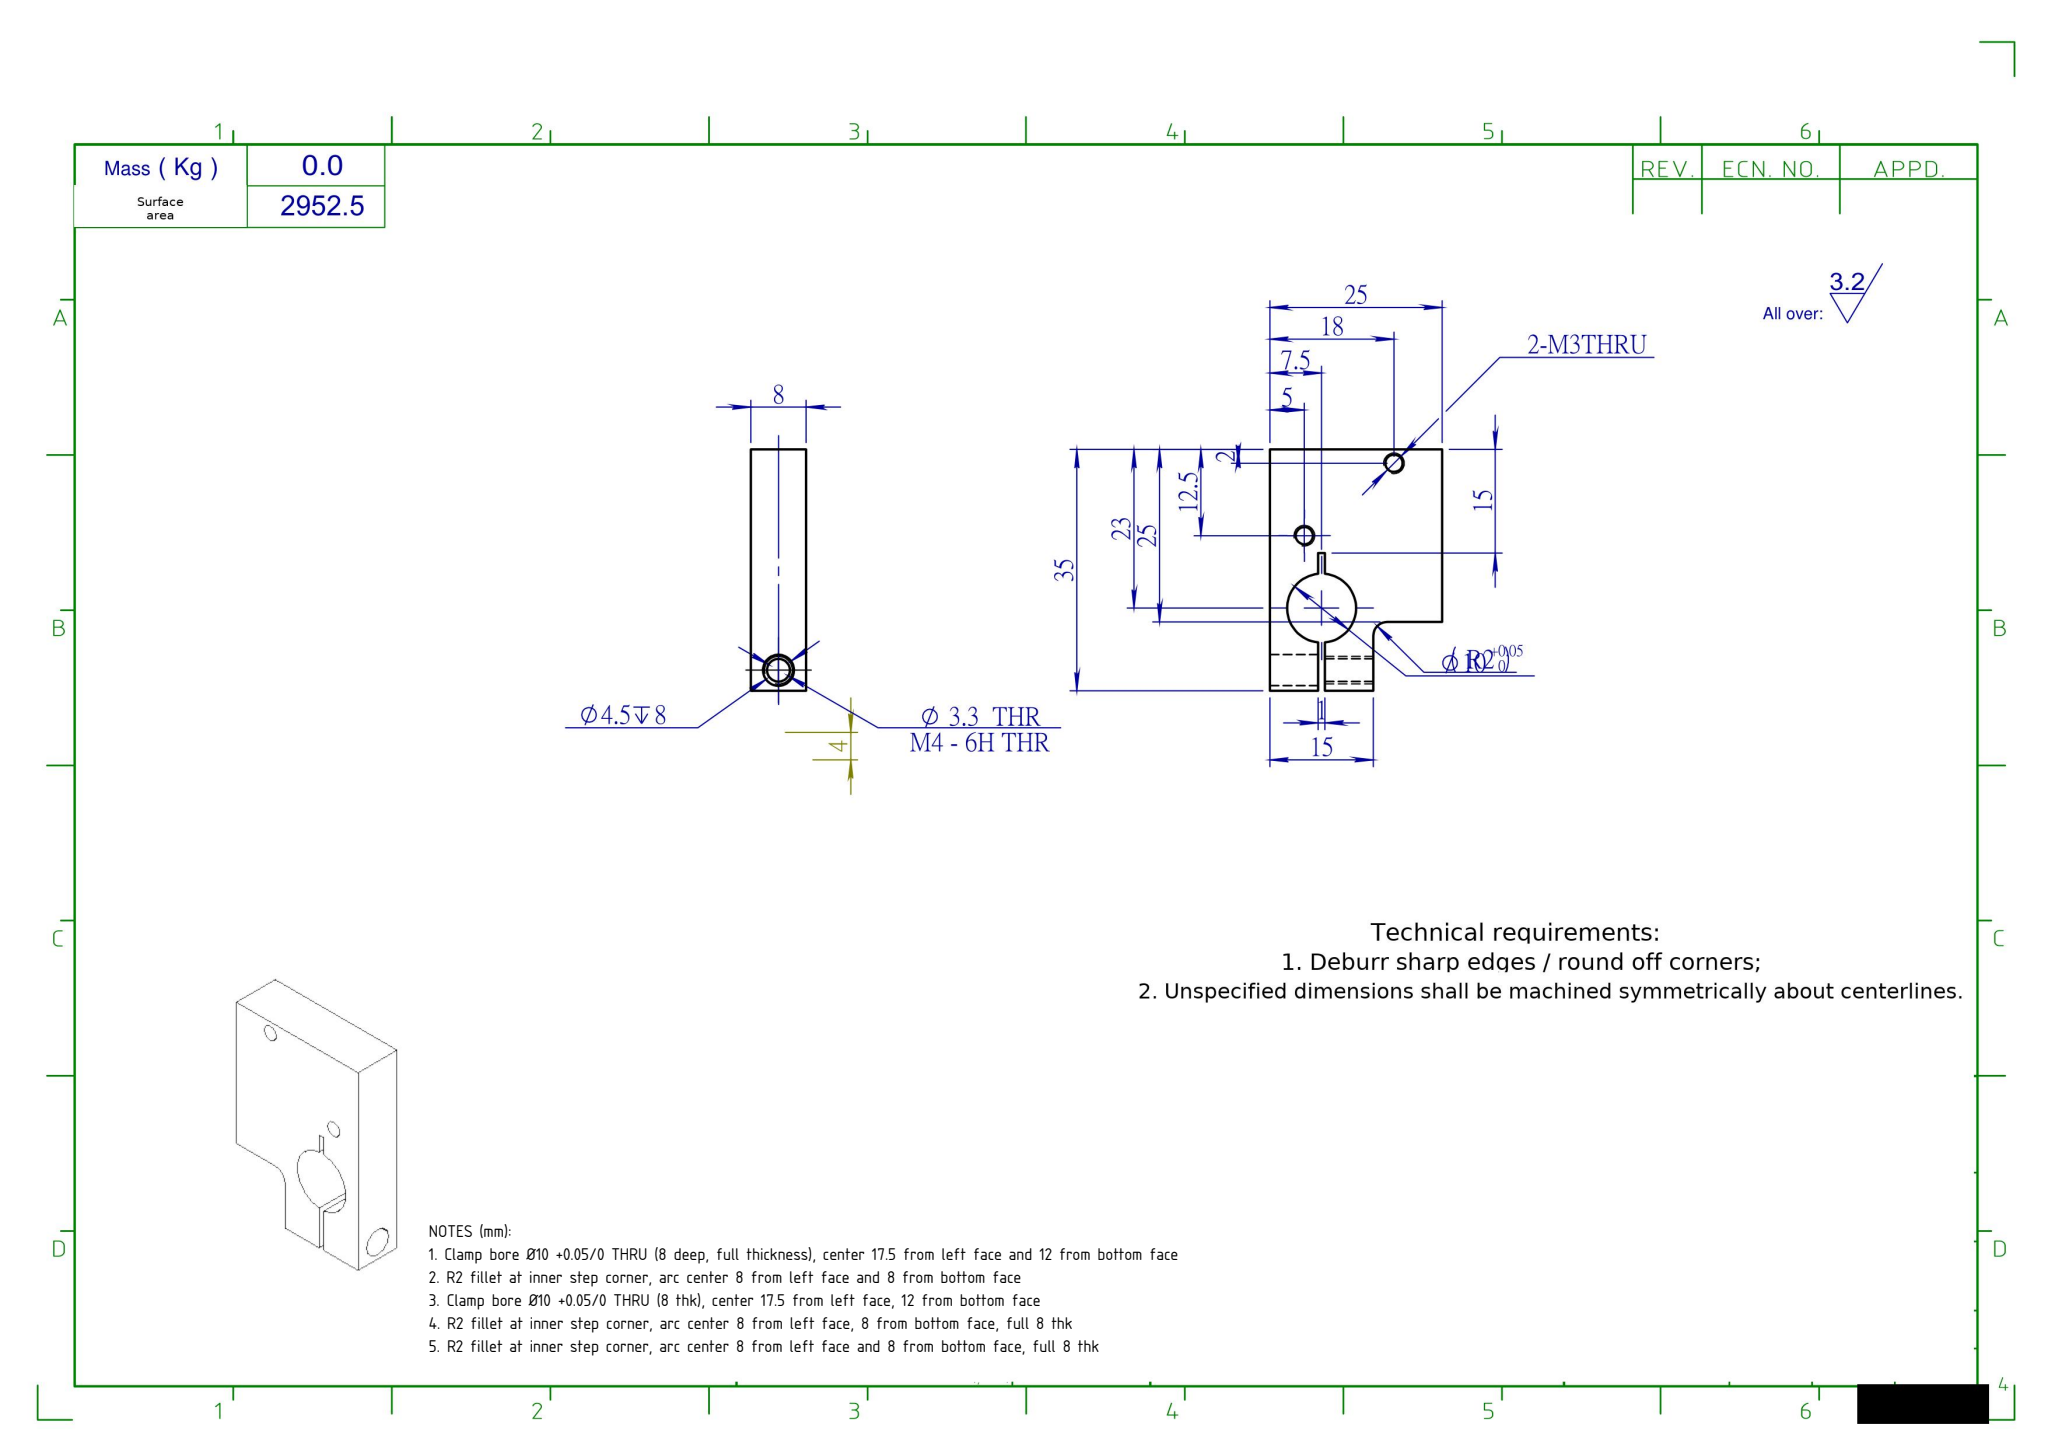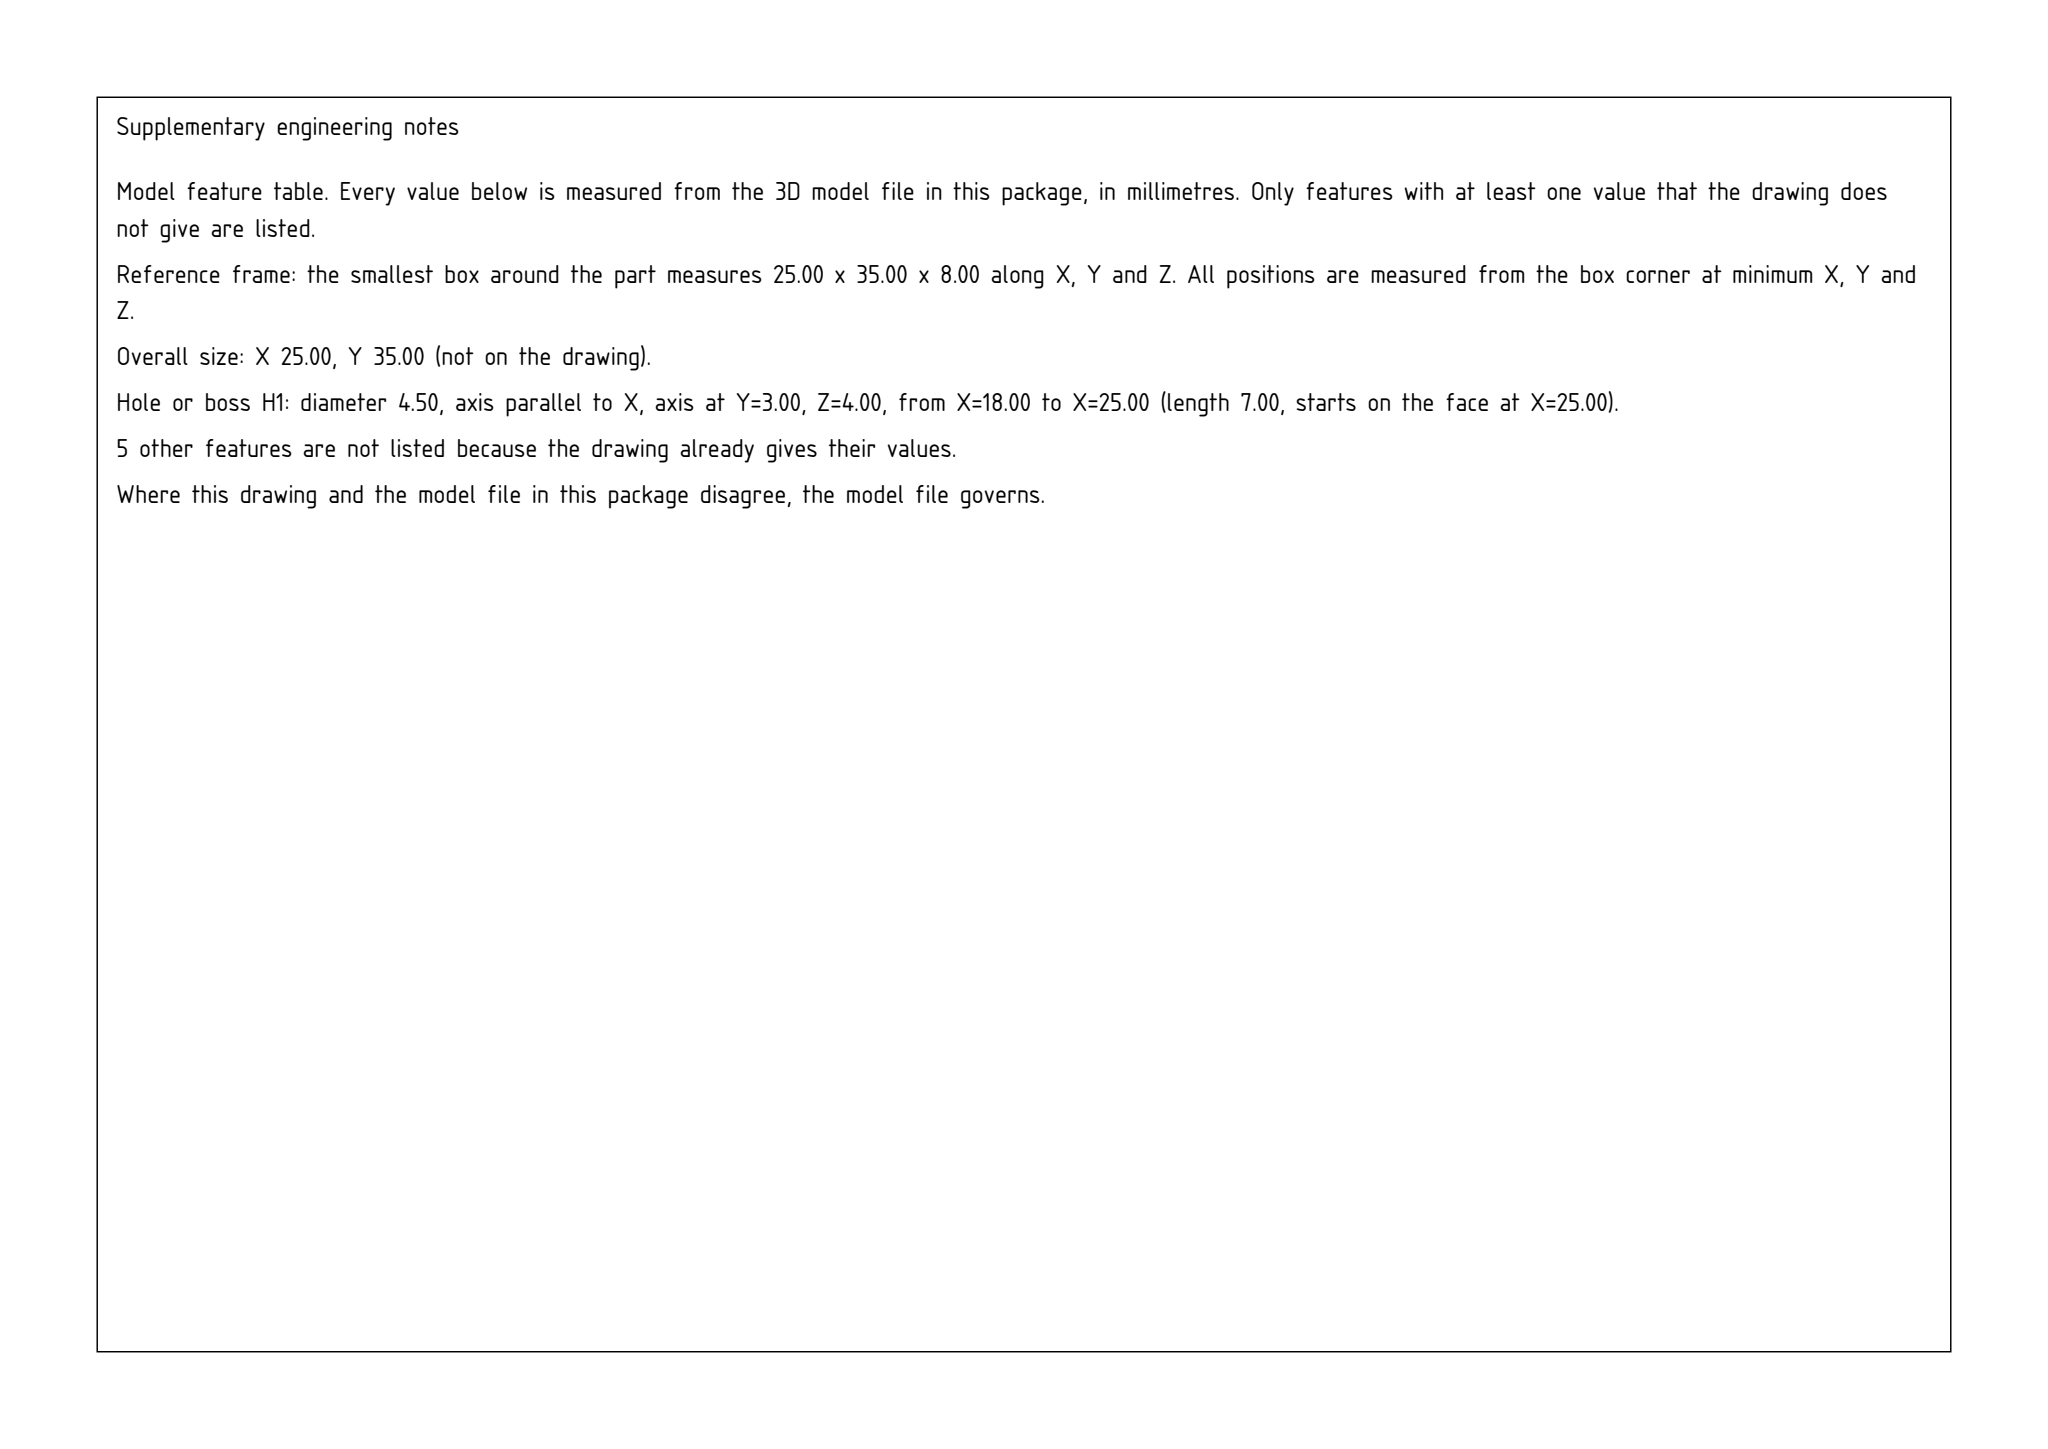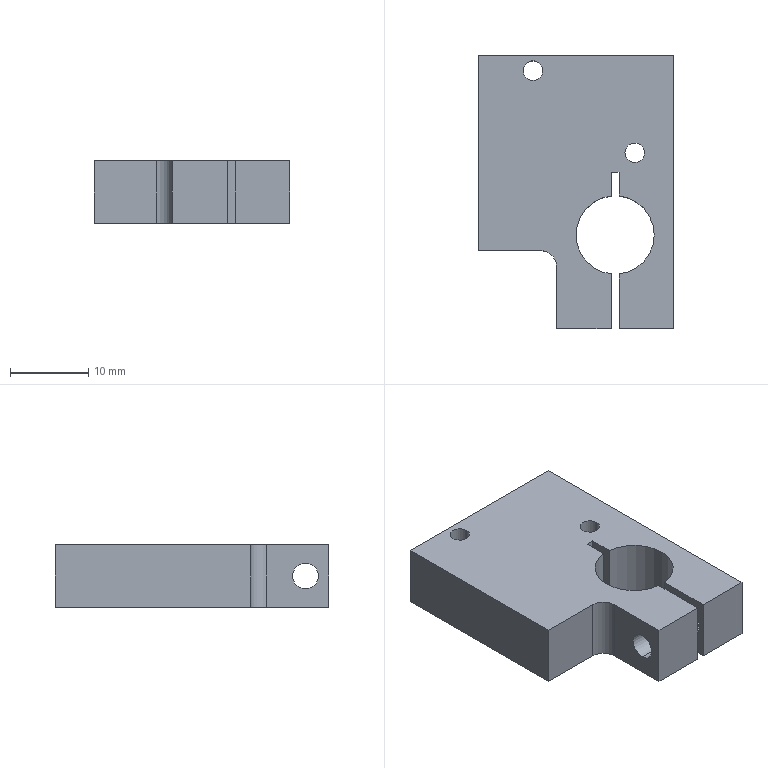Part | SolidWorks | mm | 1 solid | 26 faces | box 25 x 35 x 8 mm | volume 5249 mm3 | plane 14 | cylinder 12 | commonest cylinder face diameters 2.5 x4 10 x3 3.3 x2 4.5 x2 4 x1
Drawing notes:
Clamp bore Ø10 +0.05/0 THRU (8 deep, full thickness), center 17.5 from left face and 12 from bottom face | from the solid: cylinders: concave arc dia 10.0, axis z at [17.5, 12.0], from z0 to z8 (337° open to slot)
R2 fillet at inner step corner, arc center 8 from left face and 8 from bottom face | from the solid: cylinders: concave arc dia 4.0, axis z at [8.0, 8.0], from z0 to z8, arc 90°
Clamp bore Ø10 +0.05/0 THRU (8 thk), center 17.5 from left face, 12 from bottom face | from the solid: cylinders: concave arc dia 10.0, axis z at [17.5, 12.0], from 0.0 to 8.0
R2 fillet at inner step corner, arc center 8 from left face, 8 from bottom face, full 8 thk | from the solid: cylinders: concave arc dia 4.0 (R2), axis z at [8.0, 8.0], 90 deg, from 0.0 to 8.0
R2 fillet at inner step corner, arc center 8 from left face and 8 from bottom face, full 8 thk | from the solid: cylinders: concave arc dia 4.0 (R2), axis z at (8.0, 8.0), from 0.0 to 8.0 (90 deg)
build123d program:
from build123d import *

# Parameters (mm, degrees)
SKETCH1_W          = 15
SKETCH1_H          = 35
EXTRUDE1_DEPTH     = 8
SKETCH2_R          = 5
CUT_EXTRUDE1_DEPTH = 10
SKETCH3_W          = 1
SKETCH3_H          = 20
CUT_EXTRUDE2_DEPTH = 10
SKETCH8_W          = 8
SKETCH8_H          = 25
EXTRUDE2_DEPTH     = 10
SKETCH9_R          = 2.25
CUT_EXTRUDE3_DEPTH = 8
M4_TAPPED_HOLE1_D  = 3.3
M3_TAPPED_HOLE6_D  = 2.5
FILLET1_R          = 2


with BuildPart() as part:
    # Sketch1 → Extrude1 (new body)
    with BuildSketch(Plane.XY):
        with Locations((-14.432, 24.37)):
            Rectangle(SKETCH1_W, SKETCH1_H)
    extrude(amount=EXTRUDE1_DEPTH)

    # Sketch2 → Cut-Extrude1 (cut)
    with BuildSketch(Plane(origin=(0, 0, 0), x_dir=(-1, 0, 0), z_dir=(0, 0, -1))):
        with Locations((14.432, 18.87)):
            Circle(SKETCH2_R)
    extrude(amount=-CUT_EXTRUDE1_DEPTH, mode=Mode.SUBTRACT)

    # Sketch3 → Cut-Extrude2 (cut)
    with BuildSketch(Plane(origin=(0, 0, 0), x_dir=(-1, 0, 0), z_dir=(0, 0, -1))):
        with Locations((14.432, 16.87)):
            Rectangle(SKETCH3_W, SKETCH3_H)
    extrude(amount=-CUT_EXTRUDE2_DEPTH, mode=Mode.SUBTRACT)

    # Sketch8 → Extrude2 (add)
    with BuildSketch(Plane.ZY.offset(21.932)):
        with Locations((4, 29.37)):
            Rectangle(SKETCH8_W, SKETCH8_H)
    extrude(amount=EXTRUDE2_DEPTH)

    # Sketch9 → Cut-Extrude3 (cut)
    with BuildSketch(Plane.ZY.offset(6.932)):
        with Locations(Location((4, 9.87, 0), (0, 0, 90))):
            Circle(SKETCH9_R)
    extrude(amount=CUT_EXTRUDE3_DEPTH, mode=Mode.SUBTRACT)

    # M4 Tapped Hole1 (through all)
    with Locations(Plane(origin=(-14.932, -11.083, 0.1076), x_dir=(0, 0, 1), z_dir=(1, 0, 0))):
        with Locations((3.892, -20.953)):
            Hole(M4_TAPPED_HOLE1_D / 2)

    # M3 Tapped Hole6 (through all)
    with Locations(Plane(origin=(0, 0, 0), x_dir=(-1, 0, 0), z_dir=(0, 0, -1))):
        with Locations((11.932, 29.37), (24.932, 39.87)):
            Hole(M3_TAPPED_HOLE6_D / 2)

    # Fillet1
    fillet1_edges = [part.edges().sort_by_distance(p)[0] for p in [
        (-21.932, 16.87, 4),
    ]]
    fillet(fillet1_edges, radius=FILLET1_R)


solid = part.part
STEP:
#1=CARTESIAN_POINT('',(-13.182,29.37,8.));
#2=VERTEX_POINT('',#1);
#3=CARTESIAN_POINT('',(-10.682,29.37,8.));
#4=VERTEX_POINT('',#3);
#5=CARTESIAN_POINT('',(-11.932,29.37,8.));
#6=DIRECTION('',(0.,0.,1.));
#7=DIRECTION('',(1.,0.,0.));
#8=AXIS2_PLACEMENT_3D('',#5,#6,#7);
#9=CIRCLE('',#8,1.25);
#10=EDGE_CURVE('',#2,#4,#9,.T.);
#11=ORIENTED_EDGE('',*,*,#10,.T.);
#12=CARTESIAN_POINT('',(-10.682,29.37,-0.));
#13=VERTEX_POINT('',#12);
#14=CARTESIAN_POINT('',(-10.682,29.37,0.));
#15=DIRECTION('',(0.,0.,-1.));
#16=VECTOR('',#15,1000.);
#17=LINE('',#14,#16);
#18=EDGE_CURVE('',#4,#13,#17,.T.);
#19=ORIENTED_EDGE('',*,*,#18,.T.);
#20=CARTESIAN_POINT('',(-13.182,29.37,-0.));
#21=VERTEX_POINT('',#20);
#22=CARTESIAN_POINT('',(-11.932,29.37,-0.));
#23=DIRECTION('',(0.,0.,-1.));
#24=DIRECTION('',(-1.,0.,0.));
#25=AXIS2_PLACEMENT_3D('',#22,#23,#24);
#26=CIRCLE('',#25,1.25);
#27=EDGE_CURVE('',#13,#21,#26,.T.);
#28=ORIENTED_EDGE('',*,*,#27,.T.);
#29=CARTESIAN_POINT('',(-13.182,29.37,0.));
#30=DIRECTION('',(0.,0.,-1.));
#31=VECTOR('',#30,1000.);
#32=LINE('',#29,#31);
#33=EDGE_CURVE('',#2,#21,#32,.T.);
#34=ORIENTED_EDGE('',*,*,#33,.F.);
#35=EDGE_LOOP('',(#11,#19,#28,#34));
#36=FACE_OUTER_BOUND('',#35,.T.);
#37=CARTESIAN_POINT('',(-11.932,29.37,0.));
#38=DIRECTION('',(0.,0.,-1.));
#39=DIRECTION('',(-1.,0.,0.));
#40=AXIS2_PLACEMENT_3D('',#37,#38,#39);
#41=CYLINDRICAL_SURFACE('',#40,1.25);
#42=ADVANCED_FACE('',(#36),#41,.F.);
#43=CARTESIAN_POINT('',(-26.182,39.87,8.));
#44=VERTEX_POINT('',#43);
#45=CARTESIAN_POINT('',(-23.682,39.87,8.));
#46=VERTEX_POINT('',#45);
#47=CARTESIAN_POINT('',(-24.932,39.87,8.));
#48=DIRECTION('',(0.,0.,1.));
#49=DIRECTION('',(1.,0.,0.));
#50=AXIS2_PLACEMENT_3D('',#47,#48,#49);
#51=CIRCLE('',#50,1.25);
#52=EDGE_CURVE('',#44,#46,#51,.T.);
#53=ORIENTED_EDGE('',*,*,#52,.T.);
#54=CARTESIAN_POINT('',(-23.682,39.87,-0.));
#55=VERTEX_POINT('',#54);
#56=CARTESIAN_POINT('',(-23.682,39.87,0.));
#57=DIRECTION('',(0.,0.,-1.));
#58=VECTOR('',#57,1000.);
#59=LINE('',#56,#58);
#60=EDGE_CURVE('',#46,#55,#59,.T.);
#61=ORIENTED_EDGE('',*,*,#60,.T.);
#62=CARTESIAN_POINT('',(-26.182,39.87,-0.));
#63=VERTEX_POINT('',#62);
#64=CARTESIAN_POINT('',(-24.932,39.87,-0.));
#65=DIRECTION('',(0.,0.,-1.));
#66=DIRECTION('',(-1.,0.,0.));
#67=AXIS2_PLACEMENT_3D('',#64,#65,#66);
#68=CIRCLE('',#67,1.25);
#69=EDGE_CURVE('',#55,#63,#68,.T.);
#70=ORIENTED_EDGE('',*,*,#69,.T.);
#71=CARTESIAN_POINT('',(-26.182,39.87,0.));
#72=DIRECTION('',(0.,0.,-1.));
#73=VECTOR('',#72,1000.);
#74=LINE('',#71,#73);
#75=EDGE_CURVE('',#44,#63,#74,.T.);
#76=ORIENTED_EDGE('',*,*,#75,.F.);
#77=EDGE_LOOP('',(#53,#61,#70,#76));
#78=FACE_OUTER_BOUND('',#77,.T.);
#79=CARTESIAN_POINT('',(-24.932,39.87,0.));
#80=DIRECTION('',(0.,0.,-1.));
#81=DIRECTION('',(-1.,0.,0.));
#82=AXIS2_PLACEMENT_3D('',#79,#80,#81);
#83=CYLINDRICAL_SURFACE('',#82,1.25);
#84=ADVANCED_FACE('',(#78),#83,.F.);
#85=CARTESIAN_POINT('',(-21.932,9.87,5.65));
#86=VERTEX_POINT('',#85);
#87=CARTESIAN_POINT('',(-21.932,9.87,2.35));
#88=VERTEX_POINT('',#87);
#89=CARTESIAN_POINT('',(-21.932,9.87,4.));
#90=DIRECTION('',(1.,0.,0.));
#91=DIRECTION('',(0.,1.,0.));
#92=AXIS2_PLACEMENT_3D('',#89,#90,#91);
#93=CIRCLE('',#92,1.65);
#94=EDGE_CURVE('',#86,#88,#93,.T.);
#95=ORIENTED_EDGE('',*,*,#94,.F.);
#96=CARTESIAN_POINT('',(-14.932,9.87,5.65));
#97=VERTEX_POINT('',#96);
#98=CARTESIAN_POINT('',(-14.932,9.87,5.65));
#99=DIRECTION('',(1.,0.,0.));
#100=VECTOR('',#99,1000.);
#101=LINE('',#98,#100);
#102=EDGE_CURVE('',#86,#97,#101,.T.);
#103=ORIENTED_EDGE('',*,*,#102,.T.);
#104=CARTESIAN_POINT('',(-14.932,9.87,2.35));
#105=VERTEX_POINT('',#104);
#106=CARTESIAN_POINT('',(-14.932,9.87,4.));
#107=DIRECTION('',(1.,0.,0.));
#108=DIRECTION('',(0.,0.,-1.));
#109=AXIS2_PLACEMENT_3D('',#106,#107,#108);
#110=CIRCLE('',#109,1.65);
#111=EDGE_CURVE('',#97,#105,#110,.T.);
#112=ORIENTED_EDGE('',*,*,#111,.T.);
#113=CARTESIAN_POINT('',(-14.932,9.87,2.35));
#114=DIRECTION('',(1.,0.,0.));
#115=VECTOR('',#114,1000.);
#116=LINE('',#113,#115);
#117=EDGE_CURVE('',#88,#105,#116,.T.);
#118=ORIENTED_EDGE('',*,*,#117,.F.);
#119=EDGE_LOOP('',(#95,#103,#112,#118));
#120=FACE_OUTER_BOUND('',#119,.T.);
#121=CARTESIAN_POINT('',(-14.932,9.87,4.));
#122=DIRECTION('',(1.,0.,0.));
#123=DIRECTION('',(0.,0.,-1.));
#124=AXIS2_PLACEMENT_3D('',#121,#122,#123);
#125=CYLINDRICAL_SURFACE('',#124,1.65);
#126=ADVANCED_FACE('',(#120),#125,.F.);
#127=CARTESIAN_POINT('',(-13.932,12.12,4.));
#128=VERTEX_POINT('',#127);
#129=CARTESIAN_POINT('',(-13.932,7.62,4.));
#130=VERTEX_POINT('',#129);
#131=CARTESIAN_POINT('',(-13.932,9.87,4.));
#132=DIRECTION('',(-1.,0.,0.));
#133=DIRECTION('',(0.,1.,0.));
#134=AXIS2_PLACEMENT_3D('',#131,#132,#133);
#135=CIRCLE('',#134,2.25);
#136=EDGE_CURVE('',#128,#130,#135,.T.);
#137=ORIENTED_EDGE('',*,*,#136,.T.);
#138=CARTESIAN_POINT('',(-6.932,7.62,4.));
#139=VERTEX_POINT('',#138);
#140=CARTESIAN_POINT('',(-14.932,7.62,4.));
#141=DIRECTION('',(1.,0.,0.));
#142=VECTOR('',#141,1000.);
#143=LINE('',#140,#142);
#144=EDGE_CURVE('',#130,#139,#143,.T.);
#145=ORIENTED_EDGE('',*,*,#144,.T.);
#146=CARTESIAN_POINT('',(-6.932,12.12,4.));
#147=VERTEX_POINT('',#146);
#148=CARTESIAN_POINT('',(-6.932,9.87,4.));
#149=DIRECTION('',(-1.,-0.,0.));
#150=DIRECTION('',(0.,-1.,0.));
#151=AXIS2_PLACEMENT_3D('',#148,#149,#150);
#152=CIRCLE('',#151,2.25);
#153=EDGE_CURVE('',#147,#139,#152,.T.);
#154=ORIENTED_EDGE('',*,*,#153,.F.);
#155=CARTESIAN_POINT('',(-14.932,12.12,4.));
#156=DIRECTION('',(1.,0.,0.));
#157=VECTOR('',#156,1000.);
#158=LINE('',#155,#157);
#159=EDGE_CURVE('',#128,#147,#158,.T.);
#160=ORIENTED_EDGE('',*,*,#159,.F.);
#161=EDGE_LOOP('',(#137,#145,#154,#160));
#162=FACE_OUTER_BOUND('',#161,.T.);
#163=CARTESIAN_POINT('',(-14.932,9.87,4.));
#164=DIRECTION('',(1.,0.,0.));
#165=DIRECTION('',(0.,1.,0.));
#166=AXIS2_PLACEMENT_3D('',#163,#164,#165);
#167=CYLINDRICAL_SURFACE('',#166,2.25);
#168=ADVANCED_FACE('',(#162),#167,.F.);
#169=CARTESIAN_POINT('',(-14.932,23.845,8.));
#170=VERTEX_POINT('',#169);
#171=CARTESIAN_POINT('',(-19.432,18.87,8.));
#172=VERTEX_POINT('',#171);
#173=CARTESIAN_POINT('',(-14.432,18.87,8.));
#174=DIRECTION('',(0.,0.,1.));
#175=DIRECTION('',(1.,0.,0.));
#176=AXIS2_PLACEMENT_3D('',#173,#174,#175);
#177=CIRCLE('',#176,5.);
#178=EDGE_CURVE('',#170,#172,#177,.T.);
#179=ORIENTED_EDGE('',*,*,#178,.T.);
#180=CARTESIAN_POINT('',(-19.432,18.87,0.));
#181=VERTEX_POINT('',#180);
#182=CARTESIAN_POINT('',(-19.432,18.87,10.));
#183=DIRECTION('',(0.,0.,-1.));
#184=VECTOR('',#183,1000.);
#185=LINE('',#182,#184);
#186=EDGE_CURVE('',#172,#181,#185,.T.);
#187=ORIENTED_EDGE('',*,*,#186,.T.);
#188=CARTESIAN_POINT('',(-14.932,23.845,0.));
#189=VERTEX_POINT('',#188);
#190=CARTESIAN_POINT('',(-14.432,18.87,0.));
#191=DIRECTION('',(0.,0.,-1.));
#192=DIRECTION('',(-1.,0.,0.));
#193=AXIS2_PLACEMENT_3D('',#190,#191,#192);
#194=CIRCLE('',#193,5.);
#195=EDGE_CURVE('',#181,#189,#194,.T.);
#196=ORIENTED_EDGE('',*,*,#195,.T.);
#197=CARTESIAN_POINT('',(-14.932,23.845,10.));
#198=DIRECTION('',(0.,0.,1.));
#199=VECTOR('',#198,1000.);
#200=LINE('',#197,#199);
#201=EDGE_CURVE('',#189,#170,#200,.T.);
#202=ORIENTED_EDGE('',*,*,#201,.T.);
#203=EDGE_LOOP('',(#179,#187,#196,#202));
#204=FACE_OUTER_BOUND('',#203,.T.);
#205=CARTESIAN_POINT('',(-14.432,18.87,10.));
#206=DIRECTION('',(0.,0.,-1.));
#207=DIRECTION('',(-1.,0.,0.));
#208=AXIS2_PLACEMENT_3D('',#205,#206,#207);
#209=CYLINDRICAL_SURFACE('',#208,5.);
#210=ADVANCED_FACE('',(#204),#209,.F.);
#211=CARTESIAN_POINT('',(-6.932,6.87,0.));
#212=VERTEX_POINT('',#211);
#213=CARTESIAN_POINT('',(-6.932,41.87,0.));
#214=VERTEX_POINT('',#213);
#215=CARTESIAN_POINT('',(-6.932,41.87,0.));
#216=DIRECTION('',(-0.,1.,0.));
#217=VECTOR('',#216,1000.);
#218=LINE('',#215,#217);
#219=EDGE_CURVE('',#212,#214,#218,.T.);
#220=ORIENTED_EDGE('',*,*,#219,.T.);
#221=CARTESIAN_POINT('',(-6.932,41.87,8.));
#222=VERTEX_POINT('',#221);
#223=CARTESIAN_POINT('',(-6.932,41.87,8.));
#224=DIRECTION('',(0.,0.,-1.));
#225=VECTOR('',#224,1000.);
#226=LINE('',#223,#225);
#227=EDGE_CURVE('',#222,#214,#226,.T.);
#228=ORIENTED_EDGE('',*,*,#227,.F.);
#229=CARTESIAN_POINT('',(-6.932,6.87,8.));
#230=VERTEX_POINT('',#229);
#231=CARTESIAN_POINT('',(-6.932,41.87,8.));
#232=DIRECTION('',(-0.,1.,0.));
#233=VECTOR('',#232,1000.);
#234=LINE('',#231,#233);
#235=EDGE_CURVE('',#230,#222,#234,.T.);
#236=ORIENTED_EDGE('',*,*,#235,.F.);
#237=CARTESIAN_POINT('',(-6.932,6.87,8.));
#238=DIRECTION('',(0.,0.,-1.));
#239=VECTOR('',#238,1000.);
#240=LINE('',#237,#239);
#241=EDGE_CURVE('',#230,#212,#240,.T.);
#242=ORIENTED_EDGE('',*,*,#241,.T.);
#243=EDGE_LOOP('',(#220,#228,#236,#242));
#244=FACE_OUTER_BOUND('',#243,.T.);
#245=ORIENTED_EDGE('',*,*,#153,.T.);
#246=CARTESIAN_POINT('',(-6.932,9.87,4.));
#247=DIRECTION('',(-1.,-0.,0.));
#248=DIRECTION('',(0.,-1.,0.));
#249=AXIS2_PLACEMENT_3D('',#246,#247,#248);
#250=CIRCLE('',#249,2.25);
#251=EDGE_CURVE('',#139,#147,#250,.T.);
#252=ORIENTED_EDGE('',*,*,#251,.T.);
#253=EDGE_LOOP('',(#245,#252));
#254=FACE_BOUND('',#253,.T.);
#255=CARTESIAN_POINT('',(-6.932,41.87,8.));
#256=DIRECTION('',(-1.,-0.,0.));
#257=DIRECTION('',(0.,-1.,0.));
#258=AXIS2_PLACEMENT_3D('',#255,#256,#257);
#259=PLANE('',#258);
#260=ADVANCED_FACE('',(#244,#254),#259,.F.);
#261=CARTESIAN_POINT('',(-13.932,6.87,8.));
#262=VERTEX_POINT('',#261);
#263=CARTESIAN_POINT('',(-13.932,13.895,8.));
#264=VERTEX_POINT('',#263);
#265=CARTESIAN_POINT('',(-13.932,6.87,8.));
#266=DIRECTION('',(0.,1.,0.));
#267=VECTOR('',#266,1000.);
#268=LINE('',#265,#267);
#269=EDGE_CURVE('',#262,#264,#268,.T.);
#270=ORIENTED_EDGE('',*,*,#269,.T.);
#271=CARTESIAN_POINT('',(-13.932,13.895,0.));
#272=VERTEX_POINT('',#271);
#273=CARTESIAN_POINT('',(-13.932,13.895,10.));
#274=DIRECTION('',(0.,0.,1.));
#275=VECTOR('',#274,1000.);
#276=LINE('',#273,#275);
#277=EDGE_CURVE('',#272,#264,#276,.T.);
#278=ORIENTED_EDGE('',*,*,#277,.F.);
#279=CARTESIAN_POINT('',(-13.932,6.87,0.));
#280=VERTEX_POINT('',#279);
#281=CARTESIAN_POINT('',(-13.932,26.87,0.));
#282=DIRECTION('',(-0.,-1.,0.));
#283=VECTOR('',#282,1000.);
#284=LINE('',#281,#283);
#285=EDGE_CURVE('',#272,#280,#284,.T.);
#286=ORIENTED_EDGE('',*,*,#285,.T.);
#287=CARTESIAN_POINT('',(-13.932,6.87,10.));
#288=DIRECTION('',(0.,0.,-1.));
#289=VECTOR('',#288,1000.);
#290=LINE('',#287,#289);
#291=EDGE_CURVE('',#262,#280,#290,.T.);
#292=ORIENTED_EDGE('',*,*,#291,.F.);
#293=EDGE_LOOP('',(#270,#278,#286,#292));
#294=FACE_OUTER_BOUND('',#293,.T.);
#295=ORIENTED_EDGE('',*,*,#136,.F.);
#296=CARTESIAN_POINT('',(-13.932,9.87,4.));
#297=DIRECTION('',(-1.,0.,0.));
#298=DIRECTION('',(0.,1.,0.));
#299=AXIS2_PLACEMENT_3D('',#296,#297,#298);
#300=CIRCLE('',#299,2.25);
#301=EDGE_CURVE('',#130,#128,#300,.T.);
#302=ORIENTED_EDGE('',*,*,#301,.F.);
#303=EDGE_LOOP('',(#295,#302));
#304=FACE_BOUND('',#303,.T.);
#305=CARTESIAN_POINT('',(-13.932,26.87,10.));
#306=DIRECTION('',(1.,-0.,0.));
#307=DIRECTION('',(0.,1.,0.));
#308=AXIS2_PLACEMENT_3D('',#305,#306,#307);
#309=PLANE('',#308);
#310=ADVANCED_FACE('',(#294,#304),#309,.F.);
#311=CARTESIAN_POINT('',(-21.932,9.87,4.));
#312=DIRECTION('',(1.,0.,0.));
#313=DIRECTION('',(0.,1.,0.));
#314=AXIS2_PLACEMENT_3D('',#311,#312,#313);
#315=CIRCLE('',#314,1.65);
#316=EDGE_CURVE('',#88,#86,#315,.T.);
#317=ORIENTED_EDGE('',*,*,#316,.T.);
#318=ORIENTED_EDGE('',*,*,#94,.T.);
#319=EDGE_LOOP('',(#317,#318));
#320=FACE_BOUND('',#319,.T.);
#321=CARTESIAN_POINT('',(-21.932,14.87,8.));
#322=VERTEX_POINT('',#321);
#323=CARTESIAN_POINT('',(-21.932,6.87,8.));
#324=VERTEX_POINT('',#323);
#325=CARTESIAN_POINT('',(-21.932,41.87,8.));
#326=DIRECTION('',(0.,-1.,0.));
#327=VECTOR('',#326,1000.);
#328=LINE('',#325,#327);
#329=EDGE_CURVE('',#322,#324,#328,.T.);
#330=ORIENTED_EDGE('',*,*,#329,.F.);
#331=CARTESIAN_POINT('',(-21.932,14.87,0.));
#332=VERTEX_POINT('',#331);
#333=CARTESIAN_POINT('',(-21.932,14.87,0.));
#334=DIRECTION('',(0.,0.,-1.));
#335=VECTOR('',#334,1000.);
#336=LINE('',#333,#335);
#337=EDGE_CURVE('',#322,#332,#336,.T.);
#338=ORIENTED_EDGE('',*,*,#337,.T.);
#339=CARTESIAN_POINT('',(-21.932,6.87,0.));
#340=VERTEX_POINT('',#339);
#341=CARTESIAN_POINT('',(-21.932,41.87,0.));
#342=DIRECTION('',(0.,-1.,0.));
#343=VECTOR('',#342,1000.);
#344=LINE('',#341,#343);
#345=EDGE_CURVE('',#332,#340,#344,.T.);
#346=ORIENTED_EDGE('',*,*,#345,.T.);
#347=CARTESIAN_POINT('',(-21.932,6.87,8.));
#348=DIRECTION('',(0.,0.,-1.));
#349=VECTOR('',#348,1000.);
#350=LINE('',#347,#349);
#351=EDGE_CURVE('',#324,#340,#350,.T.);
#352=ORIENTED_EDGE('',*,*,#351,.F.);
#353=EDGE_LOOP('',(#330,#338,#346,#352));
#354=FACE_OUTER_BOUND('',#353,.T.);
#355=CARTESIAN_POINT('',(-21.932,41.87,8.));
#356=DIRECTION('',(1.,0.,0.));
#357=DIRECTION('',(-0.,1.,0.));
#358=AXIS2_PLACEMENT_3D('',#355,#356,#357);
#359=PLANE('',#358);
#360=ADVANCED_FACE('',(#320,#354),#359,.F.);
#361=CARTESIAN_POINT('',(-21.932,6.87,8.));
#362=DIRECTION('',(1.,0.,0.));
#363=VECTOR('',#362,1000.);
#364=LINE('',#361,#363);
#365=EDGE_CURVE('',#262,#230,#364,.T.);
#366=ORIENTED_EDGE('',*,*,#365,.F.);
#367=ORIENTED_EDGE('',*,*,#291,.T.);
#368=CARTESIAN_POINT('',(-21.932,6.87,0.));
#369=DIRECTION('',(1.,0.,0.));
#370=VECTOR('',#369,1000.);
#371=LINE('',#368,#370);
#372=EDGE_CURVE('',#280,#212,#371,.T.);
#373=ORIENTED_EDGE('',*,*,#372,.T.);
#374=ORIENTED_EDGE('',*,*,#241,.F.);
#375=EDGE_LOOP('',(#366,#367,#373,#374));
#376=FACE_OUTER_BOUND('',#375,.T.);
#377=CARTESIAN_POINT('',(-21.932,6.87,8.));
#378=DIRECTION('',(0.,1.,0.));
#379=DIRECTION('',(0.,0.,1.));
#380=AXIS2_PLACEMENT_3D('',#377,#378,#379);
#381=PLANE('',#380);
#382=ADVANCED_FACE('',(#376),#381,.F.);
#383=CARTESIAN_POINT('',(-13.932,23.845,0.));
#384=VERTEX_POINT('',#383);
#385=CARTESIAN_POINT('',(-14.432,18.87,0.));
#386=DIRECTION('',(0.,0.,-1.));
#387=DIRECTION('',(-1.,0.,0.));
#388=AXIS2_PLACEMENT_3D('',#385,#386,#387);
#389=CIRCLE('',#388,5.);
#390=EDGE_CURVE('',#384,#272,#389,.T.);
#391=ORIENTED_EDGE('',*,*,#390,.T.);
#392=ORIENTED_EDGE('',*,*,#277,.T.);
#393=CARTESIAN_POINT('',(-13.932,23.845,8.));
#394=VERTEX_POINT('',#393);
#395=CARTESIAN_POINT('',(-14.432,18.87,8.));
#396=DIRECTION('',(0.,0.,1.));
#397=DIRECTION('',(1.,0.,0.));
#398=AXIS2_PLACEMENT_3D('',#395,#396,#397);
#399=CIRCLE('',#398,5.);
#400=EDGE_CURVE('',#264,#394,#399,.T.);
#401=ORIENTED_EDGE('',*,*,#400,.T.);
#402=CARTESIAN_POINT('',(-13.932,23.845,10.));
#403=DIRECTION('',(0.,0.,-1.));
#404=VECTOR('',#403,1000.);
#405=LINE('',#402,#404);
#406=EDGE_CURVE('',#394,#384,#405,.T.);
#407=ORIENTED_EDGE('',*,*,#406,.T.);
#408=EDGE_LOOP('',(#391,#392,#401,#407));
#409=FACE_OUTER_BOUND('',#408,.T.);
#410=CARTESIAN_POINT('',(-14.432,18.87,10.));
#411=DIRECTION('',(0.,0.,-1.));
#412=DIRECTION('',(-1.,0.,0.));
#413=AXIS2_PLACEMENT_3D('',#410,#411,#412);
#414=CYLINDRICAL_SURFACE('',#413,5.);
#415=ADVANCED_FACE('',(#409),#414,.F.);
#416=CARTESIAN_POINT('',(-14.932,6.87,0.));
#417=VERTEX_POINT('',#416);
#418=CARTESIAN_POINT('',(-21.932,6.87,0.));
#419=DIRECTION('',(1.,0.,0.));
#420=VECTOR('',#419,1000.);
#421=LINE('',#418,#420);
#422=EDGE_CURVE('',#340,#417,#421,.T.);
#423=ORIENTED_EDGE('',*,*,#422,.T.);
#424=CARTESIAN_POINT('',(-14.932,6.87,8.));
#425=VERTEX_POINT('',#424);
#426=CARTESIAN_POINT('',(-14.932,6.87,10.));
#427=DIRECTION('',(0.,0.,-1.));
#428=VECTOR('',#427,1000.);
#429=LINE('',#426,#428);
#430=EDGE_CURVE('',#425,#417,#429,.T.);
#431=ORIENTED_EDGE('',*,*,#430,.F.);
#432=CARTESIAN_POINT('',(-21.932,6.87,8.));
#433=DIRECTION('',(1.,0.,0.));
#434=VECTOR('',#433,1000.);
#435=LINE('',#432,#434);
#436=EDGE_CURVE('',#324,#425,#435,.T.);
#437=ORIENTED_EDGE('',*,*,#436,.F.);
#438=ORIENTED_EDGE('',*,*,#351,.T.);
#439=EDGE_LOOP('',(#423,#431,#437,#438));
#440=FACE_OUTER_BOUND('',#439,.T.);
#441=CARTESIAN_POINT('',(-21.932,6.87,8.));
#442=DIRECTION('',(0.,1.,0.));
#443=DIRECTION('',(0.,0.,1.));
#444=AXIS2_PLACEMENT_3D('',#441,#442,#443);
#445=PLANE('',#444);
#446=ADVANCED_FACE('',(#440),#445,.F.);
#447=CARTESIAN_POINT('',(-31.932,41.87,0.));
#448=VERTEX_POINT('',#447);
#449=CARTESIAN_POINT('',(-21.932,41.87,0.));
#450=DIRECTION('',(-1.,0.,0.));
#451=VECTOR('',#450,1000.);
#452=LINE('',#449,#451);
#453=EDGE_CURVE('',#214,#448,#452,.T.);
#454=ORIENTED_EDGE('',*,*,#453,.T.);
#455=CARTESIAN_POINT('',(-31.932,41.87,8.));
#456=VERTEX_POINT('',#455);
#457=CARTESIAN_POINT('',(-31.932,41.87,0.));
#458=DIRECTION('',(0.,0.,-1.));
#459=VECTOR('',#458,1000.);
#460=LINE('',#457,#459);
#461=EDGE_CURVE('',#456,#448,#460,.T.);
#462=ORIENTED_EDGE('',*,*,#461,.F.);
#463=CARTESIAN_POINT('',(-21.932,41.87,8.));
#464=DIRECTION('',(-1.,0.,0.));
#465=VECTOR('',#464,1000.);
#466=LINE('',#463,#465);
#467=EDGE_CURVE('',#222,#456,#466,.T.);
#468=ORIENTED_EDGE('',*,*,#467,.F.);
#469=ORIENTED_EDGE('',*,*,#227,.T.);
#470=EDGE_LOOP('',(#454,#462,#468,#469));
#471=FACE_OUTER_BOUND('',#470,.T.);
#472=CARTESIAN_POINT('',(-21.932,41.87,8.));
#473=DIRECTION('',(0.,-1.,0.));
#474=DIRECTION('',(0.,0.,-1.));
#475=AXIS2_PLACEMENT_3D('',#472,#473,#474);
#476=PLANE('',#475);
#477=ADVANCED_FACE('',(#471),#476,.F.);
#478=ORIENTED_EDGE('',*,*,#10,.F.);
#479=CARTESIAN_POINT('',(-11.932,29.37,8.));
#480=DIRECTION('',(0.,0.,1.));
#481=DIRECTION('',(1.,0.,0.));
#482=AXIS2_PLACEMENT_3D('',#479,#480,#481);
#483=CIRCLE('',#482,1.25);
#484=EDGE_CURVE('',#4,#2,#483,.T.);
#485=ORIENTED_EDGE('',*,*,#484,.F.);
#486=EDGE_LOOP('',(#478,#485));
#487=FACE_BOUND('',#486,.T.);
#488=ORIENTED_EDGE('',*,*,#52,.F.);
#489=CARTESIAN_POINT('',(-24.932,39.87,8.));
#490=DIRECTION('',(0.,0.,1.));
#491=DIRECTION('',(1.,0.,0.));
#492=AXIS2_PLACEMENT_3D('',#489,#490,#491);
#493=CIRCLE('',#492,1.25);
#494=EDGE_CURVE('',#46,#44,#493,.T.);
#495=ORIENTED_EDGE('',*,*,#494,.F.);
#496=EDGE_LOOP('',(#488,#495));
#497=FACE_BOUND('',#496,.T.);
#498=ORIENTED_EDGE('',*,*,#269,.F.);
#499=ORIENTED_EDGE('',*,*,#365,.T.);
#500=ORIENTED_EDGE('',*,*,#235,.T.);
#501=ORIENTED_EDGE('',*,*,#467,.T.);
#502=CARTESIAN_POINT('',(-31.932,16.87,8.));
#503=VERTEX_POINT('',#502);
#504=CARTESIAN_POINT('',(-31.932,41.87,8.));
#505=DIRECTION('',(0.,1.,-0.));
#506=VECTOR('',#505,1000.);
#507=LINE('',#504,#506);
#508=EDGE_CURVE('',#503,#456,#507,.T.);
#509=ORIENTED_EDGE('',*,*,#508,.F.);
#510=CARTESIAN_POINT('',(-23.932,16.87,8.));
#511=VERTEX_POINT('',#510);
#512=CARTESIAN_POINT('',(-31.932,16.87,8.));
#513=DIRECTION('',(1.,0.,0.));
#514=VECTOR('',#513,1000.);
#515=LINE('',#512,#514);
#516=EDGE_CURVE('',#503,#511,#515,.T.);
#517=ORIENTED_EDGE('',*,*,#516,.T.);
#518=CARTESIAN_POINT('',(-23.932,14.87,8.));
#519=DIRECTION('',(0.,0.,-1.));
#520=DIRECTION('',(1.,-0.,0.));
#521=AXIS2_PLACEMENT_3D('',#518,#519,#520);
#522=CIRCLE('',#521,2.);
#523=EDGE_CURVE('',#511,#322,#522,.T.);
#524=ORIENTED_EDGE('',*,*,#523,.T.);
#525=ORIENTED_EDGE('',*,*,#329,.T.);
#526=ORIENTED_EDGE('',*,*,#436,.T.);
#527=CARTESIAN_POINT('',(-14.932,13.895,8.));
#528=VERTEX_POINT('',#527);
#529=CARTESIAN_POINT('',(-14.932,6.87,8.));
#530=DIRECTION('',(0.,-1.,0.));
#531=VECTOR('',#530,1000.);
#532=LINE('',#529,#531);
#533=EDGE_CURVE('',#528,#425,#532,.T.);
#534=ORIENTED_EDGE('',*,*,#533,.F.);
#535=CARTESIAN_POINT('',(-14.432,18.87,8.));
#536=DIRECTION('',(0.,0.,1.));
#537=DIRECTION('',(1.,0.,0.));
#538=AXIS2_PLACEMENT_3D('',#535,#536,#537);
#539=CIRCLE('',#538,5.);
#540=EDGE_CURVE('',#172,#528,#539,.T.);
#541=ORIENTED_EDGE('',*,*,#540,.F.);
#542=ORIENTED_EDGE('',*,*,#178,.F.);
#543=CARTESIAN_POINT('',(-14.932,26.87,8.));
#544=VERTEX_POINT('',#543);
#545=CARTESIAN_POINT('',(-14.932,6.87,8.));
#546=DIRECTION('',(0.,-1.,0.));
#547=VECTOR('',#546,1000.);
#548=LINE('',#545,#547);
#549=EDGE_CURVE('',#544,#170,#548,.T.);
#550=ORIENTED_EDGE('',*,*,#549,.F.);
#551=CARTESIAN_POINT('',(-13.932,26.87,8.));
#552=VERTEX_POINT('',#551);
#553=CARTESIAN_POINT('',(-21.932,26.87,8.));
#554=DIRECTION('',(-1.,0.,0.));
#555=VECTOR('',#554,1000.);
#556=LINE('',#553,#555);
#557=EDGE_CURVE('',#552,#544,#556,.T.);
#558=ORIENTED_EDGE('',*,*,#557,.F.);
#559=CARTESIAN_POINT('',(-13.932,6.87,8.));
#560=DIRECTION('',(0.,1.,0.));
#561=VECTOR('',#560,1000.);
#562=LINE('',#559,#561);
#563=EDGE_CURVE('',#394,#552,#562,.T.);
#564=ORIENTED_EDGE('',*,*,#563,.F.);
#565=ORIENTED_EDGE('',*,*,#400,.F.);
#566=EDGE_LOOP('',(#498,#499,#500,#501,#509,#517,#524,#525,#526,#534,#541,#542,#550,#558,#564,#565));
#567=FACE_OUTER_BOUND('',#566,.T.);
#568=CARTESIAN_POINT('',(-21.932,6.87,8.));
#569=DIRECTION('',(0.,0.,1.));
#570=DIRECTION('',(1.,0.,0.));
#571=AXIS2_PLACEMENT_3D('',#568,#569,#570);
#572=PLANE('',#571);
#573=ADVANCED_FACE('',(#487,#497,#567),#572,.T.);
#574=CARTESIAN_POINT('',(-11.932,29.37,-0.));
#575=DIRECTION('',(0.,0.,-1.));
#576=DIRECTION('',(-1.,0.,0.));
#577=AXIS2_PLACEMENT_3D('',#574,#575,#576);
#578=CIRCLE('',#577,1.25);
#579=EDGE_CURVE('',#21,#13,#578,.T.);
#580=ORIENTED_EDGE('',*,*,#579,.F.);
#581=ORIENTED_EDGE('',*,*,#27,.F.);
#582=EDGE_LOOP('',(#580,#581));
#583=FACE_BOUND('',#582,.T.);
#584=CARTESIAN_POINT('',(-24.932,39.87,-0.));
#585=DIRECTION('',(0.,0.,-1.));
#586=DIRECTION('',(-1.,0.,0.));
#587=AXIS2_PLACEMENT_3D('',#584,#585,#586);
#588=CIRCLE('',#587,1.25);
#589=EDGE_CURVE('',#63,#55,#588,.T.);
#590=ORIENTED_EDGE('',*,*,#589,.F.);
#591=ORIENTED_EDGE('',*,*,#69,.F.);
#592=EDGE_LOOP('',(#590,#591));
#593=FACE_BOUND('',#592,.T.);
#594=ORIENTED_EDGE('',*,*,#372,.F.);
#595=ORIENTED_EDGE('',*,*,#285,.F.);
#596=ORIENTED_EDGE('',*,*,#390,.F.);
#597=CARTESIAN_POINT('',(-13.932,26.87,0.));
#598=VERTEX_POINT('',#597);
#599=CARTESIAN_POINT('',(-13.932,26.87,0.));
#600=DIRECTION('',(-0.,-1.,0.));
#601=VECTOR('',#600,1000.);
#602=LINE('',#599,#601);
#603=EDGE_CURVE('',#598,#384,#602,.T.);
#604=ORIENTED_EDGE('',*,*,#603,.F.);
#605=CARTESIAN_POINT('',(-14.932,26.87,0.));
#606=VERTEX_POINT('',#605);
#607=CARTESIAN_POINT('',(-13.932,26.87,0.));
#608=DIRECTION('',(1.,0.,0.));
#609=VECTOR('',#608,1000.);
#610=LINE('',#607,#609);
#611=EDGE_CURVE('',#606,#598,#610,.T.);
#612=ORIENTED_EDGE('',*,*,#611,.F.);
#613=CARTESIAN_POINT('',(-14.932,26.87,0.));
#614=DIRECTION('',(-0.,1.,0.));
#615=VECTOR('',#614,1000.);
#616=LINE('',#613,#615);
#617=EDGE_CURVE('',#189,#606,#616,.T.);
#618=ORIENTED_EDGE('',*,*,#617,.F.);
#619=ORIENTED_EDGE('',*,*,#195,.F.);
#620=CARTESIAN_POINT('',(-14.932,13.895,0.));
#621=VERTEX_POINT('',#620);
#622=CARTESIAN_POINT('',(-14.432,18.87,0.));
#623=DIRECTION('',(0.,0.,-1.));
#624=DIRECTION('',(-1.,0.,0.));
#625=AXIS2_PLACEMENT_3D('',#622,#623,#624);
#626=CIRCLE('',#625,5.);
#627=EDGE_CURVE('',#621,#181,#626,.T.);
#628=ORIENTED_EDGE('',*,*,#627,.F.);
#629=CARTESIAN_POINT('',(-14.932,26.87,0.));
#630=DIRECTION('',(-0.,1.,0.));
#631=VECTOR('',#630,1000.);
#632=LINE('',#629,#631);
#633=EDGE_CURVE('',#417,#621,#632,.T.);
#634=ORIENTED_EDGE('',*,*,#633,.F.);
#635=ORIENTED_EDGE('',*,*,#422,.F.);
#636=ORIENTED_EDGE('',*,*,#345,.F.);
#637=CARTESIAN_POINT('',(-23.932,16.87,0.));
#638=VERTEX_POINT('',#637);
#639=CARTESIAN_POINT('',(-23.932,14.87,0.));
#640=DIRECTION('',(0.,0.,1.));
#641=DIRECTION('',(1.,0.,0.));
#642=AXIS2_PLACEMENT_3D('',#639,#640,#641);
#643=CIRCLE('',#642,2.);
#644=EDGE_CURVE('',#332,#638,#643,.T.);
#645=ORIENTED_EDGE('',*,*,#644,.T.);
#646=CARTESIAN_POINT('',(-31.932,16.87,0.));
#647=VERTEX_POINT('',#646);
#648=CARTESIAN_POINT('',(-31.932,16.87,0.));
#649=DIRECTION('',(1.,0.,0.));
#650=VECTOR('',#649,1000.);
#651=LINE('',#648,#650);
#652=EDGE_CURVE('',#647,#638,#651,.T.);
#653=ORIENTED_EDGE('',*,*,#652,.F.);
#654=CARTESIAN_POINT('',(-31.932,41.87,0.));
#655=DIRECTION('',(0.,-1.,0.));
#656=VECTOR('',#655,1000.);
#657=LINE('',#654,#656);
#658=EDGE_CURVE('',#448,#647,#657,.T.);
#659=ORIENTED_EDGE('',*,*,#658,.F.);
#660=ORIENTED_EDGE('',*,*,#453,.F.);
#661=ORIENTED_EDGE('',*,*,#219,.F.);
#662=EDGE_LOOP('',(#594,#595,#596,#604,#612,#618,#619,#628,#634,#635,#636,#645,#653,#659,#660,#661));
#663=FACE_OUTER_BOUND('',#662,.T.);
#664=CARTESIAN_POINT('',(-21.932,6.87,0.));
#665=DIRECTION('',(0.,0.,1.));
#666=DIRECTION('',(1.,0.,0.));
#667=AXIS2_PLACEMENT_3D('',#664,#665,#666);
#668=PLANE('',#667);
#669=ADVANCED_FACE('',(#583,#593,#663),#668,.F.);
#670=ORIENTED_EDGE('',*,*,#186,.F.);
#671=ORIENTED_EDGE('',*,*,#540,.T.);
#672=CARTESIAN_POINT('',(-14.932,13.895,10.));
#673=DIRECTION('',(0.,0.,-1.));
#674=VECTOR('',#673,1000.);
#675=LINE('',#672,#674);
#676=EDGE_CURVE('',#528,#621,#675,.T.);
#677=ORIENTED_EDGE('',*,*,#676,.T.);
#678=ORIENTED_EDGE('',*,*,#627,.T.);
#679=EDGE_LOOP('',(#670,#671,#677,#678));
#680=FACE_OUTER_BOUND('',#679,.T.);
#681=CARTESIAN_POINT('',(-14.432,18.87,10.));
#682=DIRECTION('',(0.,0.,-1.));
#683=DIRECTION('',(-1.,0.,0.));
#684=AXIS2_PLACEMENT_3D('',#681,#682,#683);
#685=CYLINDRICAL_SURFACE('',#684,5.);
#686=ADVANCED_FACE('',(#680),#685,.F.);
#687=CARTESIAN_POINT('',(-14.932,9.87,4.));
#688=DIRECTION('',(1.,0.,0.));
#689=DIRECTION('',(0.,0.,-1.));
#690=AXIS2_PLACEMENT_3D('',#687,#688,#689);
#691=CIRCLE('',#690,1.65);
#692=EDGE_CURVE('',#105,#97,#691,.T.);
#693=ORIENTED_EDGE('',*,*,#692,.F.);
#694=ORIENTED_EDGE('',*,*,#111,.F.);
#695=EDGE_LOOP('',(#693,#694));
#696=FACE_BOUND('',#695,.T.);
#697=ORIENTED_EDGE('',*,*,#533,.T.);
#698=ORIENTED_EDGE('',*,*,#430,.T.);
#699=ORIENTED_EDGE('',*,*,#633,.T.);
#700=ORIENTED_EDGE('',*,*,#676,.F.);
#701=EDGE_LOOP('',(#697,#698,#699,#700));
#702=FACE_OUTER_BOUND('',#701,.T.);
#703=CARTESIAN_POINT('',(-14.932,26.87,10.));
#704=DIRECTION('',(-1.,-0.,0.));
#705=DIRECTION('',(0.,-1.,0.));
#706=AXIS2_PLACEMENT_3D('',#703,#704,#705);
#707=PLANE('',#706);
#708=ADVANCED_FACE('',(#696,#702),#707,.F.);
#709=ORIENTED_EDGE('',*,*,#549,.T.);
#710=ORIENTED_EDGE('',*,*,#201,.F.);
#711=ORIENTED_EDGE('',*,*,#617,.T.);
#712=CARTESIAN_POINT('',(-14.932,26.87,10.));
#713=DIRECTION('',(0.,0.,-1.));
#714=VECTOR('',#713,1000.);
#715=LINE('',#712,#714);
#716=EDGE_CURVE('',#544,#606,#715,.T.);
#717=ORIENTED_EDGE('',*,*,#716,.F.);
#718=EDGE_LOOP('',(#709,#710,#711,#717));
#719=FACE_OUTER_BOUND('',#718,.T.);
#720=CARTESIAN_POINT('',(-14.932,26.87,10.));
#721=DIRECTION('',(-1.,-0.,0.));
#722=DIRECTION('',(0.,-1.,0.));
#723=AXIS2_PLACEMENT_3D('',#720,#721,#722);
#724=PLANE('',#723);
#725=ADVANCED_FACE('',(#719),#724,.F.);
#726=ORIENTED_EDGE('',*,*,#563,.T.);
#727=CARTESIAN_POINT('',(-13.932,26.87,10.));
#728=DIRECTION('',(0.,0.,-1.));
#729=VECTOR('',#728,1000.);
#730=LINE('',#727,#729);
#731=EDGE_CURVE('',#552,#598,#730,.T.);
#732=ORIENTED_EDGE('',*,*,#731,.T.);
#733=ORIENTED_EDGE('',*,*,#603,.T.);
#734=ORIENTED_EDGE('',*,*,#406,.F.);
#735=EDGE_LOOP('',(#726,#732,#733,#734));
#736=FACE_OUTER_BOUND('',#735,.T.);
#737=CARTESIAN_POINT('',(-13.932,26.87,10.));
#738=DIRECTION('',(1.,-0.,0.));
#739=DIRECTION('',(0.,1.,0.));
#740=AXIS2_PLACEMENT_3D('',#737,#738,#739);
#741=PLANE('',#740);
#742=ADVANCED_FACE('',(#736),#741,.F.);
#743=ORIENTED_EDGE('',*,*,#557,.T.);
#744=ORIENTED_EDGE('',*,*,#716,.T.);
#745=ORIENTED_EDGE('',*,*,#611,.T.);
#746=ORIENTED_EDGE('',*,*,#731,.F.);
#747=EDGE_LOOP('',(#743,#744,#745,#746));
#748=FACE_OUTER_BOUND('',#747,.T.);
#749=CARTESIAN_POINT('',(-13.932,26.87,10.));
#750=DIRECTION('',(0.,1.,0.));
#751=DIRECTION('',(0.,0.,1.));
#752=AXIS2_PLACEMENT_3D('',#749,#750,#751);
#753=PLANE('',#752);
#754=ADVANCED_FACE('',(#748),#753,.F.);
#755=ORIENTED_EDGE('',*,*,#652,.T.);
#756=CARTESIAN_POINT('',(-23.932,16.87,8.));
#757=DIRECTION('',(0.,0.,1.));
#758=VECTOR('',#757,1000.);
#759=LINE('',#756,#758);
#760=EDGE_CURVE('',#638,#511,#759,.T.);
#761=ORIENTED_EDGE('',*,*,#760,.T.);
#762=ORIENTED_EDGE('',*,*,#516,.F.);
#763=CARTESIAN_POINT('',(-31.932,16.87,0.));
#764=DIRECTION('',(0.,0.,1.));
#765=VECTOR('',#764,1000.);
#766=LINE('',#763,#765);
#767=EDGE_CURVE('',#647,#503,#766,.T.);
#768=ORIENTED_EDGE('',*,*,#767,.F.);
#769=EDGE_LOOP('',(#755,#761,#762,#768));
#770=FACE_OUTER_BOUND('',#769,.T.);
#771=CARTESIAN_POINT('',(-31.932,16.87,0.));
#772=DIRECTION('',(0.,1.,0.));
#773=DIRECTION('',(0.,0.,1.));
#774=AXIS2_PLACEMENT_3D('',#771,#772,#773);
#775=PLANE('',#774);
#776=ADVANCED_FACE('',(#770),#775,.F.);
#777=ORIENTED_EDGE('',*,*,#658,.T.);
#778=ORIENTED_EDGE('',*,*,#767,.T.);
#779=ORIENTED_EDGE('',*,*,#508,.T.);
#780=ORIENTED_EDGE('',*,*,#461,.T.);
#781=EDGE_LOOP('',(#777,#778,#779,#780));
#782=FACE_OUTER_BOUND('',#781,.T.);
#783=CARTESIAN_POINT('',(-31.932,16.87,0.));
#784=DIRECTION('',(-1.,0.,0.));
#785=DIRECTION('',(0.,0.,1.));
#786=AXIS2_PLACEMENT_3D('',#783,#784,#785);
#787=PLANE('',#786);
#788=ADVANCED_FACE('',(#782),#787,.T.);
#789=ORIENTED_EDGE('',*,*,#144,.F.);
#790=ORIENTED_EDGE('',*,*,#301,.T.);
#791=ORIENTED_EDGE('',*,*,#159,.T.);
#792=ORIENTED_EDGE('',*,*,#251,.F.);
#793=EDGE_LOOP('',(#789,#790,#791,#792));
#794=FACE_OUTER_BOUND('',#793,.T.);
#795=CARTESIAN_POINT('',(-14.932,9.87,4.));
#796=DIRECTION('',(1.,0.,0.));
#797=DIRECTION('',(0.,1.,0.));
#798=AXIS2_PLACEMENT_3D('',#795,#796,#797);
#799=CYLINDRICAL_SURFACE('',#798,2.25);
#800=ADVANCED_FACE('',(#794),#799,.F.);
#801=ORIENTED_EDGE('',*,*,#102,.F.);
#802=ORIENTED_EDGE('',*,*,#316,.F.);
#803=ORIENTED_EDGE('',*,*,#117,.T.);
#804=ORIENTED_EDGE('',*,*,#692,.T.);
#805=EDGE_LOOP('',(#801,#802,#803,#804));
#806=FACE_OUTER_BOUND('',#805,.T.);
#807=CARTESIAN_POINT('',(-14.932,9.87,4.));
#808=DIRECTION('',(1.,0.,0.));
#809=DIRECTION('',(0.,0.,-1.));
#810=AXIS2_PLACEMENT_3D('',#807,#808,#809);
#811=CYLINDRICAL_SURFACE('',#810,1.65);
#812=ADVANCED_FACE('',(#806),#811,.F.);
#813=ORIENTED_EDGE('',*,*,#60,.F.);
#814=ORIENTED_EDGE('',*,*,#494,.T.);
#815=ORIENTED_EDGE('',*,*,#75,.T.);
#816=ORIENTED_EDGE('',*,*,#589,.T.);
#817=EDGE_LOOP('',(#813,#814,#815,#816));
#818=FACE_OUTER_BOUND('',#817,.T.);
#819=CARTESIAN_POINT('',(-24.932,39.87,0.));
#820=DIRECTION('',(0.,0.,-1.));
#821=DIRECTION('',(-1.,0.,0.));
#822=AXIS2_PLACEMENT_3D('',#819,#820,#821);
#823=CYLINDRICAL_SURFACE('',#822,1.25);
#824=ADVANCED_FACE('',(#818),#823,.F.);
#825=ORIENTED_EDGE('',*,*,#18,.F.);
#826=ORIENTED_EDGE('',*,*,#484,.T.);
#827=ORIENTED_EDGE('',*,*,#33,.T.);
#828=ORIENTED_EDGE('',*,*,#579,.T.);
#829=EDGE_LOOP('',(#825,#826,#827,#828));
#830=FACE_OUTER_BOUND('',#829,.T.);
#831=CARTESIAN_POINT('',(-11.932,29.37,0.));
#832=DIRECTION('',(0.,0.,-1.));
#833=DIRECTION('',(-1.,0.,0.));
#834=AXIS2_PLACEMENT_3D('',#831,#832,#833);
#835=CYLINDRICAL_SURFACE('',#834,1.25);
#836=ADVANCED_FACE('',(#830),#835,.F.);
#837=ORIENTED_EDGE('',*,*,#644,.F.);
#838=ORIENTED_EDGE('',*,*,#337,.F.);
#839=ORIENTED_EDGE('',*,*,#523,.F.);
#840=ORIENTED_EDGE('',*,*,#760,.F.);
#841=EDGE_LOOP('',(#837,#838,#839,#840));
#842=FACE_OUTER_BOUND('',#841,.T.);
#843=CARTESIAN_POINT('',(-23.932,14.87,0.));
#844=DIRECTION('',(0.,0.,-1.));
#845=DIRECTION('',(-1.,0.,0.));
#846=AXIS2_PLACEMENT_3D('',#843,#844,#845);
#847=CYLINDRICAL_SURFACE('',#846,2.);
#848=ADVANCED_FACE('',(#842),#847,.F.);
#849=CLOSED_SHELL('',(#42,#84,#126,#168,#210,#260,#310,#360,#382,#415,#446,#477,#573,#669,#686,#708,#725,#742,#754,#776,#788,#800,#812,#824,#836,#848));
#850=MANIFOLD_SOLID_BREP('',#849);
#851=CARTESIAN_POINT('',(0.,0.,0.));
#852=DIRECTION('',(0.,0.,1.));
#853=DIRECTION('',(1.,0.,0.));
#854=AXIS2_PLACEMENT_3D('',#851,#852,#853);
#855=(LENGTH_UNIT()NAMED_UNIT(*)SI_UNIT(.MILLI.,.METRE.));
#856=UNCERTAINTY_MEASURE_WITH_UNIT(LENGTH_MEASURE(0.00001),#855,'','');
#857=(NAMED_UNIT(*)PLANE_ANGLE_UNIT()SI_UNIT($,.RADIAN.));
#858=(NAMED_UNIT(*)SI_UNIT($,.STERADIAN.)SOLID_ANGLE_UNIT());
#859=(GEOMETRIC_REPRESENTATION_CONTEXT(3)GLOBAL_UNCERTAINTY_ASSIGNED_CONTEXT((#856))GLOBAL_UNIT_ASSIGNED_CONTEXT((#855,#857,#858))REPRESENTATION_CONTEXT('',''));
#860=ADVANCED_BREP_SHAPE_REPRESENTATION('',(#850,#854),#859);